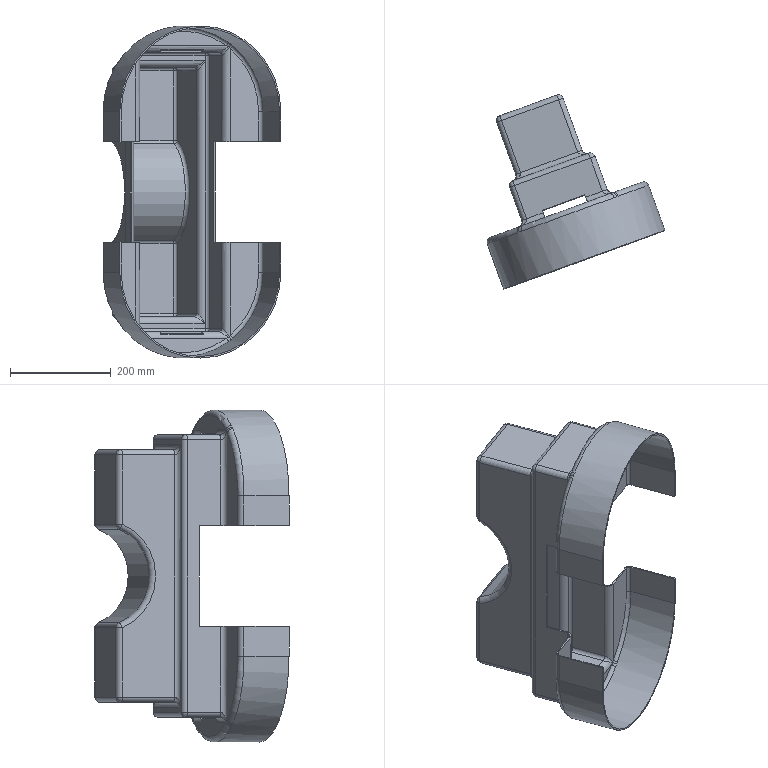Component | SolidWorks | 04-02Housing-1 | 1 solid | 206 faces | volume 1584671 mm3 | cylinder 76 | plane 58 | spline 32 | sphere 24 | torus 16 | commonest cylinder face diameters 20 x36 14 x24 26 x10 340 x2 334 x2 199.648 x1 205.648 x1